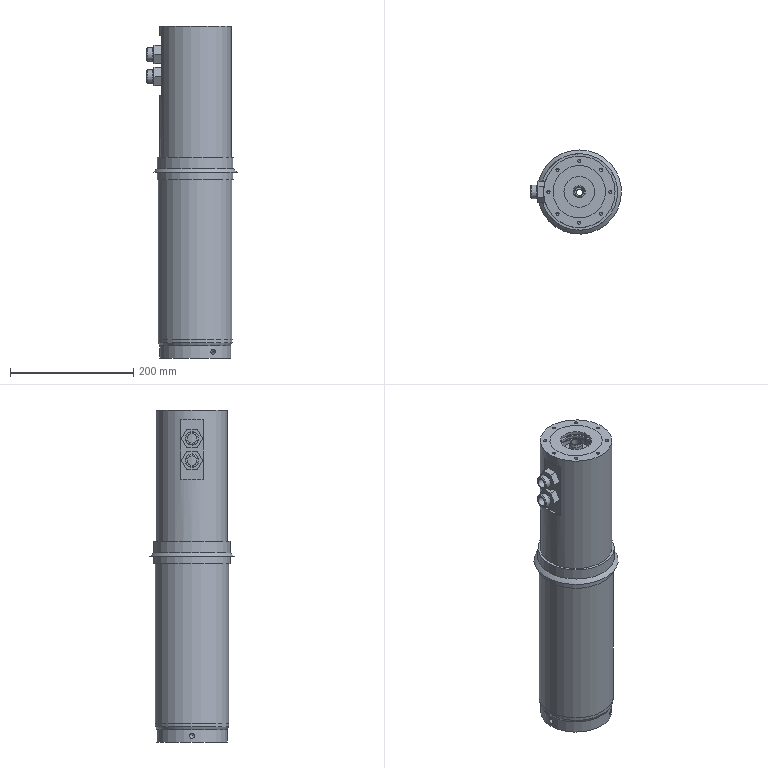Assembly | NX | mm | 18 component files | 18 solids | 291 faces | box 147.25 x 136.5 x 538 mm | volume 4135427 mm3 | cylinder 118 | plane 105 | cone 53 | sphere 9 | torus 5 | spline 1 | commonest cylinder face diameters 5 x26 85 x8 20 x8 22 x6 45 x5 95 x4 80.4 x4 30 x4
Bill of materials:
CH3404.8-4 | 1 |  | Spool-like solid of revolution: three equal-diameter outer bands separated by two recessed, smaller-diameter waists. Each band has narrow circumferential grooves. One end face has a recessed bore with internal ridges and a small central through-hole.
CH3404.8-5 | 9 |  | Solid, plain cylindrical pin-like body, roughly twice as long as its diameter. One end has a flat circular face with a conical chamfer around it. The other end is slightly domed or crowned with a small edge radius/chamfer.
CH3404.8.2-1 | 1 |  | Long thin-walled cylindrical tube with a narrow raised collar part way along its length. The upper section is very slightly smaller in diameter. One end face carries eight small holes evenly spaced around a circle.
CH3404.8-2 | 1 |  | Cylindrical sleeve with a chamfered top edge, a large central bore with internal ridges and a counterbore, three small axial holes in the top face, and small radial holes through the side wall.
CH3404.8-1 | 1 |  | Stepped cup-shaped solid of revolution. Its upper cylindrical body has two shallow circumferential grooves near the top rim. Lower down is a wider band, then an undercut groove, then a larger-diameter chamfered flange and base section with small radial holes. Inside, a cavity contains a central hollow boss with a small through-hole.
CH3404.8.2 | 1 |  | Thin flat annular ring with a tapered outer edge, giving a trapezoidal cross-section.
CH3404.8-6 | 2 |  | Hollow straight-through fitting-like body with a central hexagonal section and a cylindrical boss on each side. Each boss has chamfered ends and is joined to the hex by a short, smaller-diameter neck. There is a through-bore along the axis.
CH3404.8.1-1 | 1 |  | Short thick-walled cylindrical bushing or sleeve with an internal step (counterbore) and a chamfer on the bottom outer edge.
CH3404.8-3 | 1 |  | Long slender hollow tube with a short, slightly reduced-diameter section at each end.
Mates:
1. fix | CH3404_8_2-1 1 component
2. fix | CH3404_8-1 1 component
3. touch align | CH3404_8-2 1 face | CH3404_8-1 1 face
4. touch align | CH3404_8-2 1 face | assembly datumplane
5. touch align | CH3404_8-3 1 face | CH3404_8-1 1 face
6. touch align | CH3404_8-3 1 face | CH3404_8-1 1 face
7. touch align | CH3404_8_1 1 face | CH3404_8-1 1 face
8. touch align | CH3404_8_1 1 face | CH3404_8-2 1 face
9. touch align | CH3404_8_2 1 face | CH3404_8-1 1 face
10. touch align | CH3404_8_2 1 face | CH3404_8-1 1 face
11. touch align | CH3404_8-4 1 face | CH3404_8_2 1 face
12. parallel | CH3404_8_2 1 datumplane | assembly datumplane
13. parallel | CH3404_8-4 1 datumplane | assembly datumplane
14. touch align | CH3404_8-5 9 face | CH3404_8-2 1 face
15. touch align | CH3404_8-5 8 face | CH3404_8-2 1 face
16. touch align | CH3404_8-5 7 face | CH3404_8-2 1 face
17. touch align | CH3404_8-5 6 face | CH3404_8-2 1 face
18. touch align | CH3404_8-5 5 face | CH3404_8-2 1 face
19. touch align | CH3404_8-5 9 face | CH3404_8-1 1 face
20. touch align | CH3404_8-5 7 face | CH3404_8-1 1 face
21. touch align | CH3404_8-5 8 face | CH3404_8-1 1 face
22. touch align | CH3404_8-5 6 face | CH3404_8-1 1 face
23. touch align | CH3404_8-5 5 face | CH3404_8-1 1 face
24. touch align | CH3404_8-5 4 face | CH3404_8-2 1 face
25. touch align | CH3404_8-5 3 face | CH3404_8-2 1 face
26. touch align | CH3404_8-5 2 face | CH3404_8-2 1 face
27. touch align | CH3404_8-5 1 face | CH3404_8-2 1 face
28. touch align | CH3404_8-5 2 face | CH3404_8-1 1 face
29. touch align | CH3404_8-5 4 face | CH3404_8-1 1 face
30. touch align | CH3404_8-5 1 face | CH3404_8-1 1 face
31. touch align | CH3404_8-5 3 face | CH3404_8-1 1 face
32. touch align | CH3404_8-6 2 face | CH3404_8_2 1
33. touch align | CH3404_8-6 1 face | CH3404_8_2 1
34. touch align | CH3404_8-6 2 face | CH3404_8_2 1 face
35. touch align | CH3404_8-6 1 face | CH3404_8_2 1 face